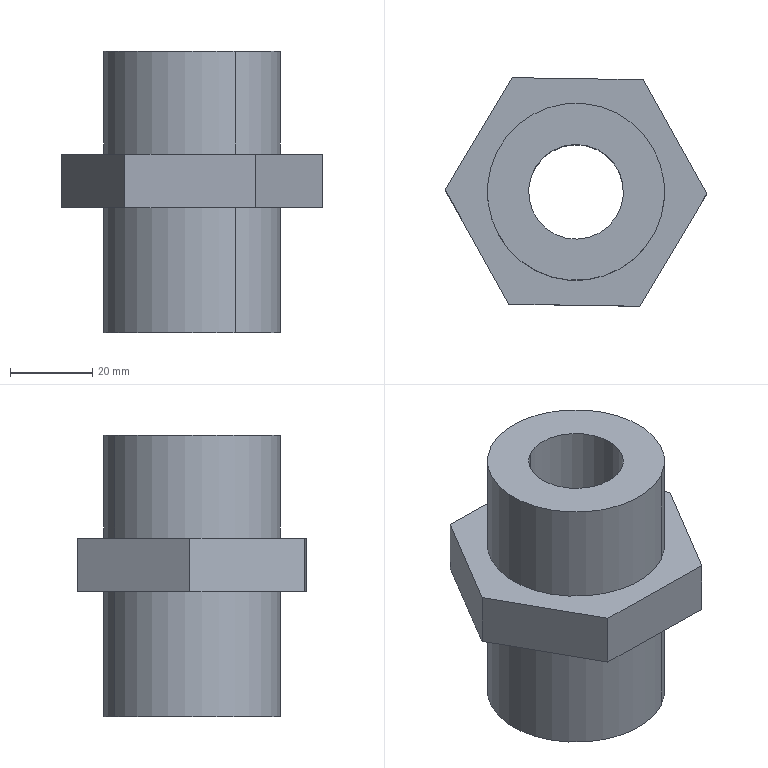Component | SolidWorks | YC1-250-04BalancerAssembly#16673-1_Rc11-4StraightInternalConnection-1 | 1 solid | 16 faces | box 63.5 x 55.49 x 68.4 mm | volume 86090 mm3 | plane 10 | cylinder 6 | commonest cylinder face diameters 43 x4 23 x2 | material Plain Carbon Steel
STEP:
#1=CARTESIAN_POINT('',(-17.698,160.776,-8.52));
#2=VERTEX_POINT('',#1);
#3=CARTESIAN_POINT('',(-18.522,162.255,-8.52));
#4=VERTEX_POINT('',#3);
#5=CARTESIAN_POINT('',(-18.11,161.516,-8.52));
#6=DIRECTION('',(0.,0.,-1.));
#7=DIRECTION('',(-0.8737,-0.4865,-0.));
#8=AXIS2_PLACEMENT_3D('',#5,#6,#7);
#9=CIRCLE('',#8,0.8465);
#10=EDGE_CURVE('',#2,#4,#9,.T.);
#11=ORIENTED_EDGE('',*,*,#10,.F.);
#12=CARTESIAN_POINT('',(-17.698,160.776,-7.323));
#13=VERTEX_POINT('',#12);
#14=CARTESIAN_POINT('',(-17.698,160.776,-8.583));
#15=DIRECTION('',(-0.,-0.,1.));
#16=VECTOR('',#15,39.37);
#17=LINE('',#14,#16);
#18=EDGE_CURVE('',#2,#13,#17,.T.);
#19=ORIENTED_EDGE('',*,*,#18,.T.);
#20=CARTESIAN_POINT('',(-18.522,162.255,-7.323));
#21=VERTEX_POINT('',#20);
#22=CARTESIAN_POINT('',(-18.11,161.516,-7.323));
#23=DIRECTION('',(0.,0.,-1.));
#24=DIRECTION('',(0.8737,0.4865,0.));
#25=AXIS2_PLACEMENT_3D('',#22,#23,#24);
#26=CIRCLE('',#25,0.8465);
#27=EDGE_CURVE('',#13,#21,#26,.T.);
#28=ORIENTED_EDGE('',*,*,#27,.T.);
#29=CARTESIAN_POINT('',(-18.522,162.255,-8.583));
#30=DIRECTION('',(-0.,-0.,1.));
#31=VECTOR('',#30,39.37);
#32=LINE('',#29,#31);
#33=EDGE_CURVE('',#4,#21,#32,.T.);
#34=ORIENTED_EDGE('',*,*,#33,.F.);
#35=EDGE_LOOP('',(#11,#19,#28,#34));
#36=FACE_OUTER_BOUND('',#35,.T.);
#37=CARTESIAN_POINT('',(-18.11,161.516,-8.583));
#38=DIRECTION('',(-0.,-0.,1.));
#39=DIRECTION('',(-0.4865,0.8737,0.));
#40=AXIS2_PLACEMENT_3D('',#37,#38,#39);
#41=CYLINDRICAL_SURFACE('',#40,0.8465);
#42=ADVANCED_FACE('',(#36),#41,.T.);
#43=CARTESIAN_POINT('',(-18.331,161.911,-8.52));
#44=VERTEX_POINT('',#43);
#45=CARTESIAN_POINT('',(-17.89,161.12,-8.52));
#46=VERTEX_POINT('',#45);
#47=CARTESIAN_POINT('',(-18.11,161.516,-8.52));
#48=DIRECTION('',(0.,0.,-1.));
#49=DIRECTION('',(-0.8737,-0.4865,0.));
#50=AXIS2_PLACEMENT_3D('',#47,#48,#49);
#51=CIRCLE('',#50,0.4528);
#52=EDGE_CURVE('',#44,#46,#51,.T.);
#53=ORIENTED_EDGE('',*,*,#52,.T.);
#54=CARTESIAN_POINT('',(-17.89,161.12,-5.827));
#55=VERTEX_POINT('',#54);
#56=CARTESIAN_POINT('',(-17.89,161.12,-8.583));
#57=DIRECTION('',(-0.,-0.,1.));
#58=VECTOR('',#57,39.37);
#59=LINE('',#56,#58);
#60=EDGE_CURVE('',#46,#55,#59,.T.);
#61=ORIENTED_EDGE('',*,*,#60,.T.);
#62=CARTESIAN_POINT('',(-18.331,161.911,-5.827));
#63=VERTEX_POINT('',#62);
#64=CARTESIAN_POINT('',(-18.11,161.516,-5.827));
#65=DIRECTION('',(0.,0.,-1.));
#66=DIRECTION('',(-0.4865,0.8737,0.));
#67=AXIS2_PLACEMENT_3D('',#64,#65,#66);
#68=CIRCLE('',#67,0.4528);
#69=EDGE_CURVE('',#63,#55,#68,.T.);
#70=ORIENTED_EDGE('',*,*,#69,.F.);
#71=CARTESIAN_POINT('',(-18.331,161.911,-8.583));
#72=DIRECTION('',(-0.,-0.,1.));
#73=VECTOR('',#72,39.37);
#74=LINE('',#71,#73);
#75=EDGE_CURVE('',#44,#63,#74,.T.);
#76=ORIENTED_EDGE('',*,*,#75,.F.);
#77=EDGE_LOOP('',(#53,#61,#70,#76));
#78=FACE_OUTER_BOUND('',#77,.T.);
#79=CARTESIAN_POINT('',(-18.11,161.516,-8.583));
#80=DIRECTION('',(-0.,-0.,1.));
#81=DIRECTION('',(-0.4865,0.8737,0.));
#82=AXIS2_PLACEMENT_3D('',#79,#80,#81);
#83=CYLINDRICAL_SURFACE('',#82,0.4528);
#84=ADVANCED_FACE('',(#78),#83,.F.);
#85=CARTESIAN_POINT('',(-18.522,162.255,-5.827));
#86=VERTEX_POINT('',#85);
#87=CARTESIAN_POINT('',(-17.698,160.776,-5.827));
#88=VERTEX_POINT('',#87);
#89=CARTESIAN_POINT('',(-18.11,161.516,-5.827));
#90=DIRECTION('',(-0.,-0.,1.));
#91=DIRECTION('',(0.4865,-0.8737,0.));
#92=AXIS2_PLACEMENT_3D('',#89,#90,#91);
#93=CIRCLE('',#92,0.8465);
#94=EDGE_CURVE('',#86,#88,#93,.T.);
#95=ORIENTED_EDGE('',*,*,#94,.F.);
#96=CARTESIAN_POINT('',(-18.522,162.255,-6.811));
#97=VERTEX_POINT('',#96);
#98=CARTESIAN_POINT('',(-18.522,162.255,-5.827));
#99=DIRECTION('',(0.,0.,-1.));
#100=VECTOR('',#99,39.37);
#101=LINE('',#98,#100);
#102=EDGE_CURVE('',#86,#97,#101,.T.);
#103=ORIENTED_EDGE('',*,*,#102,.T.);
#104=CARTESIAN_POINT('',(-17.698,160.776,-6.811));
#105=VERTEX_POINT('',#104);
#106=CARTESIAN_POINT('',(-18.11,161.516,-6.811));
#107=DIRECTION('',(-0.,-0.,1.));
#108=DIRECTION('',(0.4865,-0.8737,0.));
#109=AXIS2_PLACEMENT_3D('',#106,#107,#108);
#110=CIRCLE('',#109,0.8465);
#111=EDGE_CURVE('',#97,#105,#110,.T.);
#112=ORIENTED_EDGE('',*,*,#111,.T.);
#113=CARTESIAN_POINT('',(-17.698,160.776,-5.827));
#114=DIRECTION('',(0.,0.,-1.));
#115=VECTOR('',#114,39.37);
#116=LINE('',#113,#115);
#117=EDGE_CURVE('',#88,#105,#116,.T.);
#118=ORIENTED_EDGE('',*,*,#117,.F.);
#119=EDGE_LOOP('',(#95,#103,#112,#118));
#120=FACE_OUTER_BOUND('',#119,.T.);
#121=CARTESIAN_POINT('',(-18.11,161.516,-5.827));
#122=DIRECTION('',(0.,0.,-1.));
#123=DIRECTION('',(0.4865,-0.8737,0.));
#124=AXIS2_PLACEMENT_3D('',#121,#122,#123);
#125=CYLINDRICAL_SURFACE('',#124,0.8465);
#126=ADVANCED_FACE('',(#120),#125,.T.);
#127=ORIENTED_EDGE('',*,*,#60,.F.);
#128=CARTESIAN_POINT('',(-18.11,161.516,-8.52));
#129=DIRECTION('',(0.,0.,-1.));
#130=DIRECTION('',(-0.8737,-0.4865,0.));
#131=AXIS2_PLACEMENT_3D('',#128,#129,#130);
#132=CIRCLE('',#131,0.4528);
#133=EDGE_CURVE('',#46,#44,#132,.T.);
#134=ORIENTED_EDGE('',*,*,#133,.T.);
#135=ORIENTED_EDGE('',*,*,#75,.T.);
#136=CARTESIAN_POINT('',(-18.11,161.516,-5.827));
#137=DIRECTION('',(0.,0.,-1.));
#138=DIRECTION('',(-0.4865,0.8737,0.));
#139=AXIS2_PLACEMENT_3D('',#136,#137,#138);
#140=CIRCLE('',#139,0.4528);
#141=EDGE_CURVE('',#55,#63,#140,.T.);
#142=ORIENTED_EDGE('',*,*,#141,.F.);
#143=EDGE_LOOP('',(#127,#134,#135,#142));
#144=FACE_OUTER_BOUND('',#143,.T.);
#145=CARTESIAN_POINT('',(-18.11,161.516,-8.583));
#146=DIRECTION('',(-0.,-0.,1.));
#147=DIRECTION('',(-0.4865,0.8737,0.));
#148=AXIS2_PLACEMENT_3D('',#145,#146,#147);
#149=CYLINDRICAL_SURFACE('',#148,0.4528);
#150=ADVANCED_FACE('',(#144),#149,.F.);
#151=CARTESIAN_POINT('',(-18.11,161.516,-5.827));
#152=DIRECTION('',(-0.,-0.,1.));
#153=DIRECTION('',(0.4865,-0.8737,0.));
#154=AXIS2_PLACEMENT_3D('',#151,#152,#153);
#155=CIRCLE('',#154,0.8465);
#156=EDGE_CURVE('',#88,#86,#155,.T.);
#157=ORIENTED_EDGE('',*,*,#156,.T.);
#158=ORIENTED_EDGE('',*,*,#94,.T.);
#159=EDGE_LOOP('',(#157,#158));
#160=FACE_OUTER_BOUND('',#159,.T.);
#161=ORIENTED_EDGE('',*,*,#69,.T.);
#162=ORIENTED_EDGE('',*,*,#141,.T.);
#163=EDGE_LOOP('',(#161,#162));
#164=FACE_BOUND('',#163,.T.);
#165=CARTESIAN_POINT('',(-18.11,161.516,-5.827));
#166=DIRECTION('',(-0.,-0.,1.));
#167=DIRECTION('',(-0.4865,0.8737,-0.));
#168=AXIS2_PLACEMENT_3D('',#165,#166,#167);
#169=PLANE('',#168);
#170=ADVANCED_FACE('',(#160,#164),#169,.T.);
#171=ORIENTED_EDGE('',*,*,#102,.F.);
#172=ORIENTED_EDGE('',*,*,#156,.F.);
#173=ORIENTED_EDGE('',*,*,#117,.T.);
#174=CARTESIAN_POINT('',(-18.11,161.516,-6.811));
#175=DIRECTION('',(-0.,-0.,1.));
#176=DIRECTION('',(0.4865,-0.8737,0.));
#177=AXIS2_PLACEMENT_3D('',#174,#175,#176);
#178=CIRCLE('',#177,0.8465);
#179=EDGE_CURVE('',#105,#97,#178,.T.);
#180=ORIENTED_EDGE('',*,*,#179,.T.);
#181=EDGE_LOOP('',(#171,#172,#173,#180));
#182=FACE_OUTER_BOUND('',#181,.T.);
#183=CARTESIAN_POINT('',(-18.11,161.516,-5.827));
#184=DIRECTION('',(0.,0.,-1.));
#185=DIRECTION('',(0.4865,-0.8737,0.));
#186=AXIS2_PLACEMENT_3D('',#183,#184,#185);
#187=CYLINDRICAL_SURFACE('',#186,0.8465);
#188=ADVANCED_FACE('',(#182),#187,.T.);
#189=ORIENTED_EDGE('',*,*,#179,.F.);
#190=ORIENTED_EDGE('',*,*,#111,.F.);
#191=EDGE_LOOP('',(#189,#190));
#192=FACE_BOUND('',#191,.T.);
#193=CARTESIAN_POINT('',(-19.36,161.535,-6.811));
#194=VERTEX_POINT('',#193);
#195=CARTESIAN_POINT('',(-18.752,160.443,-6.811));
#196=VERTEX_POINT('',#195);
#197=CARTESIAN_POINT('',(-18.752,160.443,-6.811));
#198=DIRECTION('',(0.4865,-0.8737,0.));
#199=VECTOR('',#198,39.37);
#200=LINE('',#197,#199);
#201=EDGE_CURVE('',#194,#196,#200,.T.);
#202=ORIENTED_EDGE('',*,*,#201,.T.);
#203=CARTESIAN_POINT('',(-17.502,160.424,-6.811));
#204=VERTEX_POINT('',#203);
#205=CARTESIAN_POINT('',(-18.752,160.443,-6.811));
#206=DIRECTION('',(0.9999,-0.01552,0.));
#207=VECTOR('',#206,39.37);
#208=LINE('',#205,#207);
#209=EDGE_CURVE('',#196,#204,#208,.T.);
#210=ORIENTED_EDGE('',*,*,#209,.T.);
#211=CARTESIAN_POINT('',(-16.86,161.496,-6.811));
#212=VERTEX_POINT('',#211);
#213=CARTESIAN_POINT('',(-17.502,160.424,-6.811));
#214=DIRECTION('',(0.5134,0.8582,0.));
#215=VECTOR('',#214,39.37);
#216=LINE('',#213,#215);
#217=EDGE_CURVE('',#204,#212,#216,.T.);
#218=ORIENTED_EDGE('',*,*,#217,.T.);
#219=CARTESIAN_POINT('',(-17.468,162.589,-6.811));
#220=VERTEX_POINT('',#219);
#221=CARTESIAN_POINT('',(-16.86,161.496,-6.811));
#222=DIRECTION('',(-0.4865,0.8737,-0.));
#223=VECTOR('',#222,39.37);
#224=LINE('',#221,#223);
#225=EDGE_CURVE('',#212,#220,#224,.T.);
#226=ORIENTED_EDGE('',*,*,#225,.T.);
#227=CARTESIAN_POINT('',(-18.718,162.608,-6.811));
#228=VERTEX_POINT('',#227);
#229=CARTESIAN_POINT('',(-17.468,162.589,-6.811));
#230=DIRECTION('',(-0.9999,0.01552,-0.));
#231=VECTOR('',#230,39.37);
#232=LINE('',#229,#231);
#233=EDGE_CURVE('',#220,#228,#232,.T.);
#234=ORIENTED_EDGE('',*,*,#233,.T.);
#235=CARTESIAN_POINT('',(-18.718,162.608,-6.811));
#236=DIRECTION('',(-0.5134,-0.8582,-0.));
#237=VECTOR('',#236,39.37);
#238=LINE('',#235,#237);
#239=EDGE_CURVE('',#228,#194,#238,.T.);
#240=ORIENTED_EDGE('',*,*,#239,.T.);
#241=EDGE_LOOP('',(#202,#210,#218,#226,#234,#240));
#242=FACE_OUTER_BOUND('',#241,.T.);
#243=CARTESIAN_POINT('',(-16.86,161.496,-6.811));
#244=DIRECTION('',(-0.,-0.,1.));
#245=DIRECTION('',(-0.4865,0.8737,-0.));
#246=AXIS2_PLACEMENT_3D('',#243,#244,#245);
#247=PLANE('',#246);
#248=ADVANCED_FACE('',(#192,#242),#247,.T.);
#249=CARTESIAN_POINT('',(-17.502,160.424,-7.323));
#250=VERTEX_POINT('',#249);
#251=CARTESIAN_POINT('',(-17.502,160.424,-6.811));
#252=DIRECTION('',(-0.,-0.,1.));
#253=VECTOR('',#252,39.37);
#254=LINE('',#251,#253);
#255=EDGE_CURVE('',#250,#204,#254,.T.);
#256=ORIENTED_EDGE('',*,*,#255,.F.);
#257=CARTESIAN_POINT('',(-16.86,161.496,-7.323));
#258=VERTEX_POINT('',#257);
#259=CARTESIAN_POINT('',(-17.502,160.424,-7.323));
#260=DIRECTION('',(0.5134,0.8582,0.));
#261=VECTOR('',#260,39.37);
#262=LINE('',#259,#261);
#263=EDGE_CURVE('',#250,#258,#262,.T.);
#264=ORIENTED_EDGE('',*,*,#263,.T.);
#265=CARTESIAN_POINT('',(-16.86,161.496,-6.811));
#266=DIRECTION('',(0.,0.,-1.));
#267=VECTOR('',#266,39.37);
#268=LINE('',#265,#267);
#269=EDGE_CURVE('',#212,#258,#268,.T.);
#270=ORIENTED_EDGE('',*,*,#269,.F.);
#271=ORIENTED_EDGE('',*,*,#217,.F.);
#272=EDGE_LOOP('',(#256,#264,#270,#271));
#273=FACE_OUTER_BOUND('',#272,.T.);
#274=CARTESIAN_POINT('',(-17.502,160.424,-6.811));
#275=DIRECTION('',(-0.8582,0.5134,-0.));
#276=DIRECTION('',(-0.5134,-0.8582,-0.));
#277=AXIS2_PLACEMENT_3D('',#274,#275,#276);
#278=PLANE('',#277);
#279=ADVANCED_FACE('',(#273),#278,.F.);
#280=CARTESIAN_POINT('',(-18.752,160.443,-7.323));
#281=VERTEX_POINT('',#280);
#282=CARTESIAN_POINT('',(-18.752,160.443,-6.811));
#283=DIRECTION('',(-0.,-0.,1.));
#284=VECTOR('',#283,39.37);
#285=LINE('',#282,#284);
#286=EDGE_CURVE('',#281,#196,#285,.T.);
#287=ORIENTED_EDGE('',*,*,#286,.F.);
#288=CARTESIAN_POINT('',(-18.752,160.443,-7.323));
#289=DIRECTION('',(0.9999,-0.01552,0.));
#290=VECTOR('',#289,39.37);
#291=LINE('',#288,#290);
#292=EDGE_CURVE('',#281,#250,#291,.T.);
#293=ORIENTED_EDGE('',*,*,#292,.T.);
#294=ORIENTED_EDGE('',*,*,#255,.T.);
#295=ORIENTED_EDGE('',*,*,#209,.F.);
#296=EDGE_LOOP('',(#287,#293,#294,#295));
#297=FACE_OUTER_BOUND('',#296,.T.);
#298=CARTESIAN_POINT('',(-18.752,160.443,-6.811));
#299=DIRECTION('',(0.01552,0.9999,0.));
#300=DIRECTION('',(-0.9999,0.01552,-0.));
#301=AXIS2_PLACEMENT_3D('',#298,#299,#300);
#302=PLANE('',#301);
#303=ADVANCED_FACE('',(#297),#302,.F.);
#304=CARTESIAN_POINT('',(-19.36,161.535,-7.323));
#305=VERTEX_POINT('',#304);
#306=CARTESIAN_POINT('',(-19.36,161.535,-6.811));
#307=DIRECTION('',(-0.,-0.,1.));
#308=VECTOR('',#307,39.37);
#309=LINE('',#306,#308);
#310=EDGE_CURVE('',#305,#194,#309,.T.);
#311=ORIENTED_EDGE('',*,*,#310,.F.);
#312=CARTESIAN_POINT('',(-19.36,161.535,-7.323));
#313=DIRECTION('',(0.4865,-0.8737,0.));
#314=VECTOR('',#313,39.37);
#315=LINE('',#312,#314);
#316=EDGE_CURVE('',#305,#281,#315,.T.);
#317=ORIENTED_EDGE('',*,*,#316,.T.);
#318=ORIENTED_EDGE('',*,*,#286,.T.);
#319=ORIENTED_EDGE('',*,*,#201,.F.);
#320=EDGE_LOOP('',(#311,#317,#318,#319));
#321=FACE_OUTER_BOUND('',#320,.T.);
#322=CARTESIAN_POINT('',(-19.36,161.535,-6.811));
#323=DIRECTION('',(0.8737,0.4865,0.));
#324=DIRECTION('',(-0.4865,0.8737,-0.));
#325=AXIS2_PLACEMENT_3D('',#322,#323,#324);
#326=PLANE('',#325);
#327=ADVANCED_FACE('',(#321),#326,.F.);
#328=CARTESIAN_POINT('',(-18.718,162.608,-7.323));
#329=VERTEX_POINT('',#328);
#330=CARTESIAN_POINT('',(-18.718,162.608,-6.811));
#331=DIRECTION('',(-0.,-0.,1.));
#332=VECTOR('',#331,39.37);
#333=LINE('',#330,#332);
#334=EDGE_CURVE('',#329,#228,#333,.T.);
#335=ORIENTED_EDGE('',*,*,#334,.F.);
#336=CARTESIAN_POINT('',(-18.718,162.608,-7.323));
#337=DIRECTION('',(-0.5134,-0.8582,-0.));
#338=VECTOR('',#337,39.37);
#339=LINE('',#336,#338);
#340=EDGE_CURVE('',#329,#305,#339,.T.);
#341=ORIENTED_EDGE('',*,*,#340,.T.);
#342=ORIENTED_EDGE('',*,*,#310,.T.);
#343=ORIENTED_EDGE('',*,*,#239,.F.);
#344=EDGE_LOOP('',(#335,#341,#342,#343));
#345=FACE_OUTER_BOUND('',#344,.T.);
#346=CARTESIAN_POINT('',(-18.718,162.608,-6.811));
#347=DIRECTION('',(0.8582,-0.5134,0.));
#348=DIRECTION('',(0.5134,0.8582,0.));
#349=AXIS2_PLACEMENT_3D('',#346,#347,#348);
#350=PLANE('',#349);
#351=ADVANCED_FACE('',(#345),#350,.F.);
#352=CARTESIAN_POINT('',(-17.468,162.589,-7.323));
#353=VERTEX_POINT('',#352);
#354=CARTESIAN_POINT('',(-17.468,162.589,-6.811));
#355=DIRECTION('',(-0.,-0.,1.));
#356=VECTOR('',#355,39.37);
#357=LINE('',#354,#356);
#358=EDGE_CURVE('',#353,#220,#357,.T.);
#359=ORIENTED_EDGE('',*,*,#358,.F.);
#360=CARTESIAN_POINT('',(-17.468,162.589,-7.323));
#361=DIRECTION('',(-0.9999,0.01552,-0.));
#362=VECTOR('',#361,39.37);
#363=LINE('',#360,#362);
#364=EDGE_CURVE('',#353,#329,#363,.T.);
#365=ORIENTED_EDGE('',*,*,#364,.T.);
#366=ORIENTED_EDGE('',*,*,#334,.T.);
#367=ORIENTED_EDGE('',*,*,#233,.F.);
#368=EDGE_LOOP('',(#359,#365,#366,#367));
#369=FACE_OUTER_BOUND('',#368,.T.);
#370=CARTESIAN_POINT('',(-17.468,162.589,-6.811));
#371=DIRECTION('',(-0.01552,-0.9999,-0.));
#372=DIRECTION('',(0.9999,-0.01552,0.));
#373=AXIS2_PLACEMENT_3D('',#370,#371,#372);
#374=PLANE('',#373);
#375=ADVANCED_FACE('',(#369),#374,.F.);
#376=ORIENTED_EDGE('',*,*,#269,.T.);
#377=CARTESIAN_POINT('',(-16.86,161.496,-7.323));
#378=DIRECTION('',(-0.4865,0.8737,-0.));
#379=VECTOR('',#378,39.37);
#380=LINE('',#377,#379);
#381=EDGE_CURVE('',#258,#353,#380,.T.);
#382=ORIENTED_EDGE('',*,*,#381,.T.);
#383=ORIENTED_EDGE('',*,*,#358,.T.);
#384=ORIENTED_EDGE('',*,*,#225,.F.);
#385=EDGE_LOOP('',(#376,#382,#383,#384));
#386=FACE_OUTER_BOUND('',#385,.T.);
#387=CARTESIAN_POINT('',(-16.86,161.496,-6.811));
#388=DIRECTION('',(-0.8737,-0.4865,-0.));
#389=DIRECTION('',(0.4865,-0.8737,0.));
#390=AXIS2_PLACEMENT_3D('',#387,#388,#389);
#391=PLANE('',#390);
#392=ADVANCED_FACE('',(#386),#391,.F.);
#393=CARTESIAN_POINT('',(-18.11,161.516,-8.52));
#394=DIRECTION('',(0.,0.,-1.));
#395=DIRECTION('',(-0.8737,-0.4865,-0.));
#396=AXIS2_PLACEMENT_3D('',#393,#394,#395);
#397=CIRCLE('',#396,0.8465);
#398=EDGE_CURVE('',#4,#2,#397,.T.);
#399=ORIENTED_EDGE('',*,*,#398,.T.);
#400=ORIENTED_EDGE('',*,*,#10,.T.);
#401=EDGE_LOOP('',(#399,#400));
#402=FACE_OUTER_BOUND('',#401,.T.);
#403=ORIENTED_EDGE('',*,*,#52,.F.);
#404=ORIENTED_EDGE('',*,*,#133,.F.);
#405=EDGE_LOOP('',(#403,#404));
#406=FACE_BOUND('',#405,.T.);
#407=CARTESIAN_POINT('',(-17.689,160.759,-8.52));
#408=DIRECTION('',(-0.,-0.,1.));
#409=DIRECTION('',(-0.8737,-0.4865,-0.));
#410=AXIS2_PLACEMENT_3D('',#407,#408,#409);
#411=PLANE('',#410);
#412=ADVANCED_FACE('',(#402,#406),#411,.F.);
#413=ORIENTED_EDGE('',*,*,#18,.F.);
#414=ORIENTED_EDGE('',*,*,#398,.F.);
#415=ORIENTED_EDGE('',*,*,#33,.T.);
#416=CARTESIAN_POINT('',(-18.11,161.516,-7.323));
#417=DIRECTION('',(0.,0.,-1.));
#418=DIRECTION('',(0.8737,0.4865,0.));
#419=AXIS2_PLACEMENT_3D('',#416,#417,#418);
#420=CIRCLE('',#419,0.8465);
#421=EDGE_CURVE('',#21,#13,#420,.T.);
#422=ORIENTED_EDGE('',*,*,#421,.T.);
#423=EDGE_LOOP('',(#413,#414,#415,#422));
#424=FACE_OUTER_BOUND('',#423,.T.);
#425=CARTESIAN_POINT('',(-18.11,161.516,-8.583));
#426=DIRECTION('',(-0.,-0.,1.));
#427=DIRECTION('',(-0.4865,0.8737,0.));
#428=AXIS2_PLACEMENT_3D('',#425,#426,#427);
#429=CYLINDRICAL_SURFACE('',#428,0.8465);
#430=ADVANCED_FACE('',(#424),#429,.T.);
#431=ORIENTED_EDGE('',*,*,#421,.F.);
#432=ORIENTED_EDGE('',*,*,#27,.F.);
#433=EDGE_LOOP('',(#431,#432));
#434=FACE_BOUND('',#433,.T.);
#435=ORIENTED_EDGE('',*,*,#263,.F.);
#436=ORIENTED_EDGE('',*,*,#292,.F.);
#437=ORIENTED_EDGE('',*,*,#316,.F.);
#438=ORIENTED_EDGE('',*,*,#340,.F.);
#439=ORIENTED_EDGE('',*,*,#364,.F.);
#440=ORIENTED_EDGE('',*,*,#381,.F.);
#441=EDGE_LOOP('',(#435,#436,#437,#438,#439,#440));
#442=FACE_OUTER_BOUND('',#441,.T.);
#443=CARTESIAN_POINT('',(-17.344,160.14,-7.323));
#444=DIRECTION('',(-0.,-0.,1.));
#445=DIRECTION('',(-0.8737,-0.4865,-0.));
#446=AXIS2_PLACEMENT_3D('',#443,#444,#445);
#447=PLANE('',#446);
#448=ADVANCED_FACE('',(#434,#442),#447,.F.);
#449=CLOSED_SHELL('',(#42,#84,#126,#150,#170,#188,#248,#279,#303,#327,#351,#375,#392,#412,#430,#448));
#450=MANIFOLD_SOLID_BREP('',#449);
#451=CARTESIAN_POINT('',(0.,0.,0.));
#452=DIRECTION('',(0.,0.,1.));
#453=DIRECTION('',(1.,0.,0.));
#454=AXIS2_PLACEMENT_3D('',#451,#452,#453);
#455=(LENGTH_UNIT()NAMED_UNIT(*)SI_UNIT($,.METRE.));
#456=LENGTH_MEASURE_WITH_UNIT(LENGTH_MEASURE(0.0254),#455);
#457=DIMENSIONAL_EXPONENTS(1.,0.,0.,0.,0.,0.,0.);
#458=(CONVERSION_BASED_UNIT('',#456)LENGTH_UNIT()NAMED_UNIT(#457));
#459=UNCERTAINTY_MEASURE_WITH_UNIT(LENGTH_MEASURE(0.00001),#458,'','');
#460=(NAMED_UNIT(*)PLANE_ANGLE_UNIT()SI_UNIT($,.RADIAN.));
#461=(NAMED_UNIT(*)SI_UNIT($,.STERADIAN.)SOLID_ANGLE_UNIT());
#462=(GEOMETRIC_REPRESENTATION_CONTEXT(3)GLOBAL_UNCERTAINTY_ASSIGNED_CONTEXT((#459))GLOBAL_UNIT_ASSIGNED_CONTEXT((#458,#460,#461))REPRESENTATION_CONTEXT('',''));
#463=ADVANCED_BREP_SHAPE_REPRESENTATION('',(#450,#454),#462);
#464=COLOUR_RGB('',0.7922,0.8196,0.9333);
#465=FILL_AREA_STYLE_COLOUR('',#464);
#466=FILL_AREA_STYLE('',(#465));
#467=SURFACE_STYLE_FILL_AREA(#466);
#468=SURFACE_SIDE_STYLE('',(#467));
#469=SURFACE_STYLE_USAGE(.BOTH.,#468);
#470=PRESENTATION_STYLE_ASSIGNMENT((#469));
#471=STYLED_ITEM('',(#470),#450);
#472=(LENGTH_UNIT()NAMED_UNIT(*)SI_UNIT($,.METRE.));
#473=LENGTH_MEASURE_WITH_UNIT(LENGTH_MEASURE(0.0254),#472);
#474=DIMENSIONAL_EXPONENTS(1.,0.,0.,0.,0.,0.,0.);
#475=(CONVERSION_BASED_UNIT('',#473)LENGTH_UNIT()NAMED_UNIT(#474));
#476=UNCERTAINTY_MEASURE_WITH_UNIT(LENGTH_MEASURE(0.00001),#475,'','');
#477=(NAMED_UNIT(*)PLANE_ANGLE_UNIT()SI_UNIT($,.RADIAN.));
#478=(NAMED_UNIT(*)SI_UNIT($,.STERADIAN.)SOLID_ANGLE_UNIT());
#479=(GEOMETRIC_REPRESENTATION_CONTEXT(3)GLOBAL_UNCERTAINTY_ASSIGNED_CONTEXT((#476))GLOBAL_UNIT_ASSIGNED_CONTEXT((#475,#477,#478))REPRESENTATION_CONTEXT('',''));
#480=MECHANICAL_DESIGN_GEOMETRIC_PRESENTATION_REPRESENTATION('',(#471),#479);
#481=PRESENTATION_LAYER_ASSIGNMENT('','',(#471));